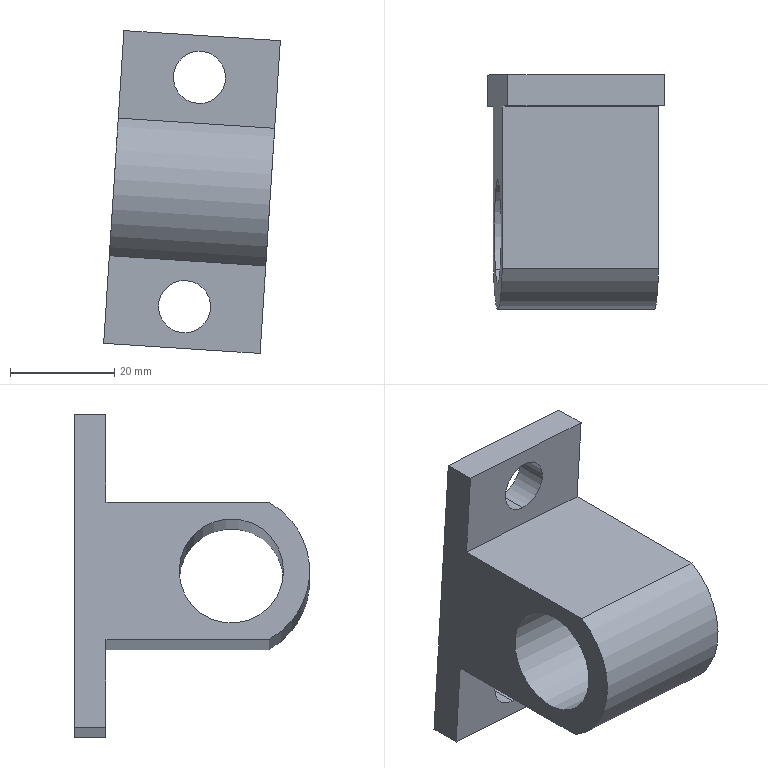Component | SolidWorks | X-AxisBallScrewSupport2-2 | 1 solid | 16 faces | box 33.82 x 45 x 61.82 mm | volume 29524 mm3 | plane 9 | cylinder 7 | commonest cylinder face diameters 10 x4 20 x2 30 x1
build123d program:
from build123d import *

# Parameters (mm, degrees)
SKETCH1_R               = 10
BOSS_EXTRUDE1_DEPTH     = 30
CUT_EXTRUDE1_DEPTH      = 832.191
CUT_EXTRUDE1_DEPTH_BACK = 832.191
CUT_EXTRUDE2_DEPTH      = 779.008
CUT_EXTRUDE2_DEPTH_BACK = 779.008
SKETCH5_R               = 5


with BuildPart() as part:
    # Sketch1 → Boss-Extrude1 (new body)
    with BuildSketch(Plane.XY):
        with BuildLine():
            Line((-298.984, -768.399), (-258.103, -724.481))
            Line((-258.103, -724.481), (-262.495, -720.393))
            Line((-262.495, -720.393), (-296.724, -711.484))
            ThreePointArc((-296.724, -711.484), (-311.482, -715.78), (-314.711, -730.807))
            Line((-314.711, -730.807), (-303.376, -764.311))
            Line((-303.376, -764.311), (-298.984, -768.399))
        make_face()
        with Locations((-300.503, -726)):
            Circle(SKETCH1_R, mode=Mode.SUBTRACT)
    extrude(amount=-BOSS_EXTRUDE1_DEPTH)

    # Sketch4 → Cut-Extrude1 (cut, two sides: drawn at the far end of the back side and taken through both)
    with BuildSketch(Plane(origin=(0, 0, -30), x_dir=(-1, 0, 0), z_dir=(0, 0, -1)).offset(-CUT_EXTRUDE1_DEPTH_BACK)):
        Polygon((314.711, -730.807), (291.929, -752.014), (303.376, -764.311), align=None)
        Polygon((296.724, -711.484), (273.942, -732.69), (262.495, -720.393), align=None)
    extrude(amount=CUT_EXTRUDE1_DEPTH + CUT_EXTRUDE1_DEPTH_BACK, mode=Mode.SUBTRACT)

    # Sketch5 → Cut-Extrude2 (cut, two sides: drawn at the far end of the back side and taken through both)
    with BuildSketch(Plane(origin=(218.636, -203.516, 0), x_dir=(0, 0, 1), z_dir=(-0.732, 0.6813, 0)).offset(-CUT_EXTRUDE2_DEPTH_BACK)):
        with Locations(Location((-15, -714.151, 0), (0, 0, 90))):
            Circle(SKETCH5_R)
        with Locations(Location((-15, -758.151, 0), (0, 0, 90))):
            Circle(SKETCH5_R)
    extrude(amount=CUT_EXTRUDE2_DEPTH + CUT_EXTRUDE2_DEPTH_BACK, mode=Mode.SUBTRACT)


solid = part.part

# Placed as in the assembly
solid = solid.moved(Location((207.979, -970.699, 434.364), (180, 86.288, -47.051)))
STEP:
#1=CARTESIAN_POINT('',(5.654,-26.22,-12.843));
#2=VERTEX_POINT('',#1);
#3=CARTESIAN_POINT('',(5.679,-26.22,-12.45));
#4=VERTEX_POINT('',#3);
#5=CARTESIAN_POINT('',(5.666,-26.22,-12.647));
#6=DIRECTION('',(0.,1.,0.));
#7=DIRECTION('',(0.06474,-0.,0.9979));
#8=AXIS2_PLACEMENT_3D('',#5,#6,#7);
#9=CIRCLE('',#8,0.1969);
#10=EDGE_CURVE('',#2,#4,#9,.T.);
#11=ORIENTED_EDGE('',*,*,#10,.T.);
#12=CARTESIAN_POINT('',(5.679,-26.457,-12.45));
#13=VERTEX_POINT('',#12);
#14=CARTESIAN_POINT('',(5.679,-25.042,-12.45));
#15=DIRECTION('',(0.,-1.,0.));
#16=VECTOR('',#15,39.37);
#17=LINE('',#14,#16);
#18=EDGE_CURVE('',#4,#13,#17,.T.);
#19=ORIENTED_EDGE('',*,*,#18,.T.);
#20=CARTESIAN_POINT('',(5.654,-26.457,-12.843));
#21=VERTEX_POINT('',#20);
#22=CARTESIAN_POINT('',(5.666,-26.457,-12.647));
#23=DIRECTION('',(0.,1.,0.));
#24=DIRECTION('',(0.06474,-0.,0.9979));
#25=AXIS2_PLACEMENT_3D('',#22,#23,#24);
#26=CIRCLE('',#25,0.1969);
#27=EDGE_CURVE('',#21,#13,#26,.T.);
#28=ORIENTED_EDGE('',*,*,#27,.F.);
#29=CARTESIAN_POINT('',(5.654,-25.042,-12.843));
#30=DIRECTION('',(0.,-1.,0.));
#31=VECTOR('',#30,39.37);
#32=LINE('',#29,#31);
#33=EDGE_CURVE('',#2,#21,#32,.T.);
#34=ORIENTED_EDGE('',*,*,#33,.F.);
#35=EDGE_LOOP('',(#11,#19,#28,#34));
#36=FACE_OUTER_BOUND('',#35,.T.);
#37=CARTESIAN_POINT('',(5.666,-25.042,-12.647));
#38=DIRECTION('',(0.,-1.,0.));
#39=DIRECTION('',(-0.06474,0.,-0.9979));
#40=AXIS2_PLACEMENT_3D('',#37,#38,#39);
#41=CYLINDRICAL_SURFACE('',#40,0.1969);
#42=ADVANCED_FACE('',(#36),#41,.F.);
#43=CARTESIAN_POINT('',(5.766,-26.22,-11.114));
#44=VERTEX_POINT('',#43);
#45=CARTESIAN_POINT('',(5.791,-26.22,-10.722));
#46=VERTEX_POINT('',#45);
#47=CARTESIAN_POINT('',(5.779,-26.22,-10.918));
#48=DIRECTION('',(0.,1.,0.));
#49=DIRECTION('',(0.06474,-0.,0.9979));
#50=AXIS2_PLACEMENT_3D('',#47,#48,#49);
#51=CIRCLE('',#50,0.1969);
#52=EDGE_CURVE('',#44,#46,#51,.T.);
#53=ORIENTED_EDGE('',*,*,#52,.T.);
#54=CARTESIAN_POINT('',(5.791,-26.457,-10.722));
#55=VERTEX_POINT('',#54);
#56=CARTESIAN_POINT('',(5.791,-25.042,-10.722));
#57=DIRECTION('',(0.,-1.,0.));
#58=VECTOR('',#57,39.37);
#59=LINE('',#56,#58);
#60=EDGE_CURVE('',#46,#55,#59,.T.);
#61=ORIENTED_EDGE('',*,*,#60,.T.);
#62=CARTESIAN_POINT('',(5.766,-26.457,-11.114));
#63=VERTEX_POINT('',#62);
#64=CARTESIAN_POINT('',(5.779,-26.457,-10.918));
#65=DIRECTION('',(0.,1.,0.));
#66=DIRECTION('',(0.06474,0.,0.9979));
#67=AXIS2_PLACEMENT_3D('',#64,#65,#66);
#68=CIRCLE('',#67,0.1969);
#69=EDGE_CURVE('',#63,#55,#68,.T.);
#70=ORIENTED_EDGE('',*,*,#69,.F.);
#71=CARTESIAN_POINT('',(5.766,-25.042,-11.114));
#72=DIRECTION('',(0.,-1.,0.));
#73=VECTOR('',#72,39.37);
#74=LINE('',#71,#73);
#75=EDGE_CURVE('',#44,#63,#74,.T.);
#76=ORIENTED_EDGE('',*,*,#75,.F.);
#77=EDGE_LOOP('',(#53,#61,#70,#76));
#78=FACE_OUTER_BOUND('',#77,.T.);
#79=CARTESIAN_POINT('',(5.779,-25.042,-10.918));
#80=DIRECTION('',(0.,-1.,0.));
#81=DIRECTION('',(-0.06474,0.,-0.9979));
#82=AXIS2_PLACEMENT_3D('',#79,#80,#81);
#83=CYLINDRICAL_SURFACE('',#82,0.1969);
#84=ADVANCED_FACE('',(#78),#83,.F.);
#85=CARTESIAN_POINT('',(5.116,-27.69,-12.012));
#86=VERTEX_POINT('',#85);
#87=CARTESIAN_POINT('',(5.151,-27.113,-11.476));
#88=VERTEX_POINT('',#87);
#89=CARTESIAN_POINT('',(5.133,-27.402,-11.744));
#90=DIRECTION('',(0.9979,0.,-0.06474));
#91=DIRECTION('',(0.04411,0.732,0.6799));
#92=AXIS2_PLACEMENT_3D('',#89,#90,#91);
#93=CIRCLE('',#92,0.3937);
#94=EDGE_CURVE('',#86,#88,#93,.T.);
#95=ORIENTED_EDGE('',*,*,#94,.F.);
#96=CARTESIAN_POINT('',(6.294,-27.69,-12.088));
#97=VERTEX_POINT('',#96);
#98=CARTESIAN_POINT('',(5.116,-27.69,-12.012));
#99=DIRECTION('',(0.9979,0.,-0.06474));
#100=VECTOR('',#99,39.37);
#101=LINE('',#98,#100);
#102=EDGE_CURVE('',#86,#97,#101,.T.);
#103=ORIENTED_EDGE('',*,*,#102,.T.);
#104=CARTESIAN_POINT('',(6.329,-27.113,-11.553));
#105=VERTEX_POINT('',#104);
#106=CARTESIAN_POINT('',(6.312,-27.402,-11.821));
#107=DIRECTION('',(0.9979,0.,-0.06474));
#108=DIRECTION('',(0.04411,0.732,0.6799));
#109=AXIS2_PLACEMENT_3D('',#106,#107,#108);
#110=CIRCLE('',#109,0.3937);
#111=EDGE_CURVE('',#97,#105,#110,.T.);
#112=ORIENTED_EDGE('',*,*,#111,.T.);
#113=CARTESIAN_POINT('',(5.151,-27.113,-11.476));
#114=DIRECTION('',(0.9979,0.,-0.06474));
#115=VECTOR('',#114,39.37);
#116=LINE('',#113,#115);
#117=EDGE_CURVE('',#88,#105,#116,.T.);
#118=ORIENTED_EDGE('',*,*,#117,.F.);
#119=EDGE_LOOP('',(#95,#103,#112,#118));
#120=FACE_OUTER_BOUND('',#119,.T.);
#121=CARTESIAN_POINT('',(5.133,-27.402,-11.744));
#122=DIRECTION('',(0.9979,0.,-0.06474));
#123=DIRECTION('',(0.04411,0.732,0.6799));
#124=AXIS2_PLACEMENT_3D('',#121,#122,#123);
#125=CYLINDRICAL_SURFACE('',#124,0.3937);
#126=ADVANCED_FACE('',(#120),#125,.F.);
#127=CARTESIAN_POINT('',(6.235,-26.22,-12.999));
#128=VERTEX_POINT('',#127);
#129=CARTESIAN_POINT('',(6.235,-26.457,-12.999));
#130=VERTEX_POINT('',#129);
#131=CARTESIAN_POINT('',(6.235,-38.216,-12.999));
#132=DIRECTION('',(-0.,-1.,-0.));
#133=VECTOR('',#132,39.37);
#134=LINE('',#131,#133);
#135=EDGE_CURVE('',#128,#130,#134,.T.);
#136=ORIENTED_EDGE('',*,*,#135,.T.);
#137=CARTESIAN_POINT('',(5.057,-26.457,-12.923));
#138=VERTEX_POINT('',#137);
#139=CARTESIAN_POINT('',(5.057,-26.457,-12.923));
#140=DIRECTION('',(0.9979,0.,-0.06474));
#141=VECTOR('',#140,39.37);
#142=LINE('',#139,#141);
#143=EDGE_CURVE('',#138,#130,#142,.T.);
#144=ORIENTED_EDGE('',*,*,#143,.F.);
#145=CARTESIAN_POINT('',(5.057,-26.22,-12.923));
#146=VERTEX_POINT('',#145);
#147=CARTESIAN_POINT('',(5.057,-38.216,-12.923));
#148=DIRECTION('',(-0.,-1.,-0.));
#149=VECTOR('',#148,39.37);
#150=LINE('',#147,#149);
#151=EDGE_CURVE('',#146,#138,#150,.T.);
#152=ORIENTED_EDGE('',*,*,#151,.F.);
#153=CARTESIAN_POINT('',(5.057,-26.22,-12.923));
#154=DIRECTION('',(0.9979,0.,-0.06474));
#155=VECTOR('',#154,39.37);
#156=LINE('',#153,#155);
#157=EDGE_CURVE('',#146,#128,#156,.T.);
#158=ORIENTED_EDGE('',*,*,#157,.T.);
#159=EDGE_LOOP('',(#136,#144,#152,#158));
#160=FACE_OUTER_BOUND('',#159,.T.);
#161=CARTESIAN_POINT('',(5.057,-38.216,-12.923));
#162=DIRECTION('',(0.06474,-0.,0.9979));
#163=DIRECTION('',(-0.,-1.,-0.));
#164=AXIS2_PLACEMENT_3D('',#161,#162,#163);
#165=PLANE('',#164);
#166=ADVANCED_FACE('',(#160),#165,.F.);
#167=CARTESIAN_POINT('',(6.345,-27.682,-11.302));
#168=VERTEX_POINT('',#167);
#169=CARTESIAN_POINT('',(6.278,-27.682,-12.339));
#170=VERTEX_POINT('',#169);
#171=CARTESIAN_POINT('',(6.312,-27.402,-11.821));
#172=DIRECTION('',(0.9979,0.,-0.06474));
#173=DIRECTION('',(0.04411,0.732,0.6799));
#174=AXIS2_PLACEMENT_3D('',#171,#172,#173);
#175=CIRCLE('',#174,0.5906);
#176=EDGE_CURVE('',#168,#170,#175,.T.);
#177=ORIENTED_EDGE('',*,*,#176,.F.);
#178=CARTESIAN_POINT('',(5.167,-27.682,-11.226));
#179=VERTEX_POINT('',#178);
#180=CARTESIAN_POINT('',(5.167,-27.682,-11.226));
#181=DIRECTION('',(0.9979,0.,-0.06474));
#182=VECTOR('',#181,39.37);
#183=LINE('',#180,#182);
#184=EDGE_CURVE('',#179,#168,#183,.T.);
#185=ORIENTED_EDGE('',*,*,#184,.F.);
#186=CARTESIAN_POINT('',(5.1,-27.682,-12.263));
#187=VERTEX_POINT('',#186);
#188=CARTESIAN_POINT('',(5.133,-27.402,-11.744));
#189=DIRECTION('',(0.9979,0.,-0.06474));
#190=DIRECTION('',(0.04411,0.732,0.6799));
#191=AXIS2_PLACEMENT_3D('',#188,#189,#190);
#192=CIRCLE('',#191,0.5906);
#193=EDGE_CURVE('',#179,#187,#192,.T.);
#194=ORIENTED_EDGE('',*,*,#193,.T.);
#195=CARTESIAN_POINT('',(5.1,-27.682,-12.263));
#196=DIRECTION('',(0.9979,0.,-0.06474));
#197=VECTOR('',#196,39.37);
#198=LINE('',#195,#197);
#199=EDGE_CURVE('',#187,#170,#198,.T.);
#200=ORIENTED_EDGE('',*,*,#199,.T.);
#201=EDGE_LOOP('',(#177,#185,#194,#200));
#202=FACE_OUTER_BOUND('',#201,.T.);
#203=CARTESIAN_POINT('',(5.133,-27.402,-11.744));
#204=DIRECTION('',(0.9979,0.,-0.06474));
#205=DIRECTION('',(0.04411,0.732,0.6799));
#206=AXIS2_PLACEMENT_3D('',#203,#204,#205);
#207=CYLINDRICAL_SURFACE('',#206,0.5906);
#208=ADVANCED_FACE('',(#202),#207,.T.);
#209=CARTESIAN_POINT('',(6.388,-26.22,-10.642));
#210=VERTEX_POINT('',#209);
#211=CARTESIAN_POINT('',(6.388,-26.457,-10.642));
#212=VERTEX_POINT('',#211);
#213=CARTESIAN_POINT('',(6.388,-38.216,-10.642));
#214=DIRECTION('',(0.,-1.,0.));
#215=VECTOR('',#214,39.37);
#216=LINE('',#213,#215);
#217=EDGE_CURVE('',#210,#212,#216,.T.);
#218=ORIENTED_EDGE('',*,*,#217,.F.);
#219=CARTESIAN_POINT('',(5.21,-26.22,-10.565));
#220=VERTEX_POINT('',#219);
#221=CARTESIAN_POINT('',(5.21,-26.22,-10.565));
#222=DIRECTION('',(0.9979,0.,-0.06474));
#223=VECTOR('',#222,39.37);
#224=LINE('',#221,#223);
#225=EDGE_CURVE('',#220,#210,#224,.T.);
#226=ORIENTED_EDGE('',*,*,#225,.F.);
#227=CARTESIAN_POINT('',(5.21,-26.457,-10.565));
#228=VERTEX_POINT('',#227);
#229=CARTESIAN_POINT('',(5.21,-38.216,-10.565));
#230=DIRECTION('',(0.,-1.,0.));
#231=VECTOR('',#230,39.37);
#232=LINE('',#229,#231);
#233=EDGE_CURVE('',#220,#228,#232,.T.);
#234=ORIENTED_EDGE('',*,*,#233,.T.);
#235=CARTESIAN_POINT('',(5.21,-26.457,-10.565));
#236=DIRECTION('',(0.9979,0.,-0.06474));
#237=VECTOR('',#236,39.37);
#238=LINE('',#235,#237);
#239=EDGE_CURVE('',#228,#212,#238,.T.);
#240=ORIENTED_EDGE('',*,*,#239,.T.);
#241=EDGE_LOOP('',(#218,#226,#234,#240));
#242=FACE_OUTER_BOUND('',#241,.T.);
#243=CARTESIAN_POINT('',(5.21,-38.216,-10.565));
#244=DIRECTION('',(0.06474,0.,0.9979));
#245=DIRECTION('',(0.,-1.,0.));
#246=AXIS2_PLACEMENT_3D('',#243,#244,#245);
#247=PLANE('',#246);
#248=ADVANCED_FACE('',(#242),#247,.T.);
#249=ORIENTED_EDGE('',*,*,#10,.F.);
#250=CARTESIAN_POINT('',(5.666,-26.22,-12.647));
#251=DIRECTION('',(0.,1.,0.));
#252=DIRECTION('',(0.06474,-0.,0.9979));
#253=AXIS2_PLACEMENT_3D('',#250,#251,#252);
#254=CIRCLE('',#253,0.1969);
#255=EDGE_CURVE('',#4,#2,#254,.T.);
#256=ORIENTED_EDGE('',*,*,#255,.F.);
#257=EDGE_LOOP('',(#249,#256));
#258=FACE_BOUND('',#257,.T.);
#259=ORIENTED_EDGE('',*,*,#52,.F.);
#260=CARTESIAN_POINT('',(5.779,-26.22,-10.918));
#261=DIRECTION('',(0.,1.,0.));
#262=DIRECTION('',(0.06474,-0.,0.9979));
#263=AXIS2_PLACEMENT_3D('',#260,#261,#262);
#264=CIRCLE('',#263,0.1969);
#265=EDGE_CURVE('',#46,#44,#264,.T.);
#266=ORIENTED_EDGE('',*,*,#265,.F.);
#267=EDGE_LOOP('',(#259,#266));
#268=FACE_BOUND('',#267,.T.);
#269=CARTESIAN_POINT('',(8.188,-26.22,17.101));
#270=DIRECTION('',(0.06474,-0.,0.9979));
#271=VECTOR('',#270,39.37);
#272=LINE('',#269,#271);
#273=EDGE_CURVE('',#128,#210,#272,.T.);
#274=ORIENTED_EDGE('',*,*,#273,.F.);
#275=ORIENTED_EDGE('',*,*,#157,.F.);
#276=CARTESIAN_POINT('',(7.01,-26.22,17.177));
#277=DIRECTION('',(0.06474,-0.,0.9979));
#278=VECTOR('',#277,39.37);
#279=LINE('',#276,#278);
#280=EDGE_CURVE('',#146,#220,#279,.T.);
#281=ORIENTED_EDGE('',*,*,#280,.T.);
#282=ORIENTED_EDGE('',*,*,#225,.T.);
#283=EDGE_LOOP('',(#274,#275,#281,#282));
#284=FACE_OUTER_BOUND('',#283,.T.);
#285=CARTESIAN_POINT('',(7.01,-26.22,17.177));
#286=DIRECTION('',(0.,1.,0.));
#287=DIRECTION('',(0.06474,-0.,0.9979));
#288=AXIS2_PLACEMENT_3D('',#285,#286,#287);
#289=PLANE('',#288);
#290=ADVANCED_FACE('',(#258,#268,#284),#289,.T.);
#291=ORIENTED_EDGE('',*,*,#102,.F.);
#292=CARTESIAN_POINT('',(5.133,-27.402,-11.744));
#293=DIRECTION('',(0.9979,0.,-0.06474));
#294=DIRECTION('',(0.04411,0.732,0.6799));
#295=AXIS2_PLACEMENT_3D('',#292,#293,#294);
#296=CIRCLE('',#295,0.3937);
#297=EDGE_CURVE('',#88,#86,#296,.T.);
#298=ORIENTED_EDGE('',*,*,#297,.F.);
#299=ORIENTED_EDGE('',*,*,#117,.T.);
#300=CARTESIAN_POINT('',(6.312,-27.402,-11.821));
#301=DIRECTION('',(0.9979,0.,-0.06474));
#302=DIRECTION('',(0.04411,0.732,0.6799));
#303=AXIS2_PLACEMENT_3D('',#300,#301,#302);
#304=CIRCLE('',#303,0.3937);
#305=EDGE_CURVE('',#105,#97,#304,.T.);
#306=ORIENTED_EDGE('',*,*,#305,.T.);
#307=EDGE_LOOP('',(#291,#298,#299,#306));
#308=FACE_OUTER_BOUND('',#307,.T.);
#309=CARTESIAN_POINT('',(5.133,-27.402,-11.744));
#310=DIRECTION('',(0.9979,0.,-0.06474));
#311=DIRECTION('',(0.04411,0.732,0.6799));
#312=AXIS2_PLACEMENT_3D('',#309,#310,#311);
#313=CYLINDRICAL_SURFACE('',#312,0.3937);
#314=ADVANCED_FACE('',(#308),#313,.F.);
#315=CARTESIAN_POINT('',(5.167,-26.457,-11.226));
#316=VERTEX_POINT('',#315);
#317=CARTESIAN_POINT('',(5.167,-38.216,-11.226));
#318=DIRECTION('',(0.,1.,0.));
#319=VECTOR('',#318,39.37);
#320=LINE('',#317,#319);
#321=EDGE_CURVE('',#179,#316,#320,.T.);
#322=ORIENTED_EDGE('',*,*,#321,.T.);
#323=CARTESIAN_POINT('',(7.01,-26.457,17.177));
#324=DIRECTION('',(0.06474,-0.,0.9979));
#325=VECTOR('',#324,39.37);
#326=LINE('',#323,#325);
#327=EDGE_CURVE('',#316,#228,#326,.T.);
#328=ORIENTED_EDGE('',*,*,#327,.T.);
#329=ORIENTED_EDGE('',*,*,#233,.F.);
#330=ORIENTED_EDGE('',*,*,#280,.F.);
#331=ORIENTED_EDGE('',*,*,#151,.T.);
#332=CARTESIAN_POINT('',(5.1,-26.457,-12.263));
#333=VERTEX_POINT('',#332);
#334=CARTESIAN_POINT('',(7.01,-26.457,17.177));
#335=DIRECTION('',(0.06474,-0.,0.9979));
#336=VECTOR('',#335,39.37);
#337=LINE('',#334,#336);
#338=EDGE_CURVE('',#138,#333,#337,.T.);
#339=ORIENTED_EDGE('',*,*,#338,.T.);
#340=CARTESIAN_POINT('',(5.1,-38.216,-12.263));
#341=DIRECTION('',(-0.,-1.,-0.));
#342=VECTOR('',#341,39.37);
#343=LINE('',#340,#342);
#344=EDGE_CURVE('',#333,#187,#343,.T.);
#345=ORIENTED_EDGE('',*,*,#344,.T.);
#346=ORIENTED_EDGE('',*,*,#193,.F.);
#347=EDGE_LOOP('',(#322,#328,#329,#330,#331,#339,#345,#346));
#348=FACE_OUTER_BOUND('',#347,.T.);
#349=ORIENTED_EDGE('',*,*,#297,.T.);
#350=ORIENTED_EDGE('',*,*,#94,.T.);
#351=EDGE_LOOP('',(#349,#350));
#352=FACE_BOUND('',#351,.T.);
#353=CARTESIAN_POINT('',(7.01,-38.216,17.177));
#354=DIRECTION('',(0.9979,0.,-0.06474));
#355=DIRECTION('',(0.04411,0.732,0.6799));
#356=AXIS2_PLACEMENT_3D('',#353,#354,#355);
#357=PLANE('',#356);
#358=ADVANCED_FACE('',(#348,#352),#357,.F.);
#359=CARTESIAN_POINT('',(6.345,-26.457,-11.302));
#360=VERTEX_POINT('',#359);
#361=CARTESIAN_POINT('',(6.388,-26.457,-10.642));
#362=DIRECTION('',(-0.06474,0.,-0.9979));
#363=VECTOR('',#362,39.37);
#364=LINE('',#361,#363);
#365=EDGE_CURVE('',#212,#360,#364,.T.);
#366=ORIENTED_EDGE('',*,*,#365,.T.);
#367=CARTESIAN_POINT('',(6.345,-27.682,-11.302));
#368=DIRECTION('',(-0.,-1.,-0.));
#369=VECTOR('',#368,39.37);
#370=LINE('',#367,#369);
#371=EDGE_CURVE('',#360,#168,#370,.T.);
#372=ORIENTED_EDGE('',*,*,#371,.T.);
#373=ORIENTED_EDGE('',*,*,#176,.T.);
#374=CARTESIAN_POINT('',(6.278,-26.457,-12.339));
#375=VERTEX_POINT('',#374);
#376=CARTESIAN_POINT('',(6.278,-27.682,-12.339));
#377=DIRECTION('',(0.,1.,0.));
#378=VECTOR('',#377,39.37);
#379=LINE('',#376,#378);
#380=EDGE_CURVE('',#170,#375,#379,.T.);
#381=ORIENTED_EDGE('',*,*,#380,.T.);
#382=CARTESIAN_POINT('',(6.278,-26.457,-12.339));
#383=DIRECTION('',(-0.06474,0.,-0.9979));
#384=VECTOR('',#383,39.37);
#385=LINE('',#382,#384);
#386=EDGE_CURVE('',#375,#130,#385,.T.);
#387=ORIENTED_EDGE('',*,*,#386,.T.);
#388=ORIENTED_EDGE('',*,*,#135,.F.);
#389=ORIENTED_EDGE('',*,*,#273,.T.);
#390=ORIENTED_EDGE('',*,*,#217,.T.);
#391=EDGE_LOOP('',(#366,#372,#373,#381,#387,#388,#389,#390));
#392=FACE_OUTER_BOUND('',#391,.T.);
#393=ORIENTED_EDGE('',*,*,#305,.F.);
#394=ORIENTED_EDGE('',*,*,#111,.F.);
#395=EDGE_LOOP('',(#393,#394));
#396=FACE_BOUND('',#395,.T.);
#397=CARTESIAN_POINT('',(8.188,-38.216,17.101));
#398=DIRECTION('',(0.9979,0.,-0.06474));
#399=DIRECTION('',(0.04411,0.732,0.6799));
#400=AXIS2_PLACEMENT_3D('',#397,#398,#399);
#401=PLANE('',#400);
#402=ADVANCED_FACE('',(#392,#396),#401,.T.);
#403=ORIENTED_EDGE('',*,*,#27,.T.);
#404=CARTESIAN_POINT('',(5.666,-26.457,-12.647));
#405=DIRECTION('',(0.,1.,0.));
#406=DIRECTION('',(0.06474,-0.,0.9979));
#407=AXIS2_PLACEMENT_3D('',#404,#405,#406);
#408=CIRCLE('',#407,0.1969);
#409=EDGE_CURVE('',#13,#21,#408,.T.);
#410=ORIENTED_EDGE('',*,*,#409,.T.);
#411=EDGE_LOOP('',(#403,#410));
#412=FACE_BOUND('',#411,.T.);
#413=ORIENTED_EDGE('',*,*,#143,.T.);
#414=ORIENTED_EDGE('',*,*,#386,.F.);
#415=CARTESIAN_POINT('',(6.278,-26.457,-12.339));
#416=DIRECTION('',(-0.9979,-0.,0.06474));
#417=VECTOR('',#416,39.37);
#418=LINE('',#415,#417);
#419=EDGE_CURVE('',#375,#333,#418,.T.);
#420=ORIENTED_EDGE('',*,*,#419,.T.);
#421=ORIENTED_EDGE('',*,*,#338,.F.);
#422=EDGE_LOOP('',(#413,#414,#420,#421));
#423=FACE_OUTER_BOUND('',#422,.T.);
#424=CARTESIAN_POINT('',(6.278,-26.457,-12.339));
#425=DIRECTION('',(0.,1.,0.));
#426=DIRECTION('',(0.06474,-0.,0.9979));
#427=AXIS2_PLACEMENT_3D('',#424,#425,#426);
#428=PLANE('',#427);
#429=ADVANCED_FACE('',(#412,#423),#428,.F.);
#430=ORIENTED_EDGE('',*,*,#419,.F.);
#431=ORIENTED_EDGE('',*,*,#380,.F.);
#432=ORIENTED_EDGE('',*,*,#199,.F.);
#433=ORIENTED_EDGE('',*,*,#344,.F.);
#434=EDGE_LOOP('',(#430,#431,#432,#433));
#435=FACE_OUTER_BOUND('',#434,.T.);
#436=CARTESIAN_POINT('',(6.278,-27.682,-12.339));
#437=DIRECTION('',(0.06474,-0.,0.9979));
#438=DIRECTION('',(-0.,-1.,-0.));
#439=AXIS2_PLACEMENT_3D('',#436,#437,#438);
#440=PLANE('',#439);
#441=ADVANCED_FACE('',(#435),#440,.F.);
#442=ORIENTED_EDGE('',*,*,#69,.T.);
#443=CARTESIAN_POINT('',(5.779,-26.457,-10.918));
#444=DIRECTION('',(0.,1.,0.));
#445=DIRECTION('',(0.06474,0.,0.9979));
#446=AXIS2_PLACEMENT_3D('',#443,#444,#445);
#447=CIRCLE('',#446,0.1969);
#448=EDGE_CURVE('',#55,#63,#447,.T.);
#449=ORIENTED_EDGE('',*,*,#448,.T.);
#450=EDGE_LOOP('',(#442,#449));
#451=FACE_BOUND('',#450,.T.);
#452=CARTESIAN_POINT('',(6.345,-26.457,-11.302));
#453=DIRECTION('',(-0.9979,-0.,0.06474));
#454=VECTOR('',#453,39.37);
#455=LINE('',#452,#454);
#456=EDGE_CURVE('',#360,#316,#455,.T.);
#457=ORIENTED_EDGE('',*,*,#456,.F.);
#458=ORIENTED_EDGE('',*,*,#365,.F.);
#459=ORIENTED_EDGE('',*,*,#239,.F.);
#460=ORIENTED_EDGE('',*,*,#327,.F.);
#461=EDGE_LOOP('',(#457,#458,#459,#460));
#462=FACE_OUTER_BOUND('',#461,.T.);
#463=CARTESIAN_POINT('',(6.388,-26.457,-10.642));
#464=DIRECTION('',(0.,1.,0.));
#465=DIRECTION('',(0.06474,-0.,0.9979));
#466=AXIS2_PLACEMENT_3D('',#463,#464,#465);
#467=PLANE('',#466);
#468=ADVANCED_FACE('',(#451,#462),#467,.F.);
#469=ORIENTED_EDGE('',*,*,#184,.T.);
#470=ORIENTED_EDGE('',*,*,#371,.F.);
#471=ORIENTED_EDGE('',*,*,#456,.T.);
#472=ORIENTED_EDGE('',*,*,#321,.F.);
#473=EDGE_LOOP('',(#469,#470,#471,#472));
#474=FACE_OUTER_BOUND('',#473,.T.);
#475=CARTESIAN_POINT('',(6.345,-27.682,-11.302));
#476=DIRECTION('',(-0.06474,0.,-0.9979));
#477=DIRECTION('',(0.,1.,0.));
#478=AXIS2_PLACEMENT_3D('',#475,#476,#477);
#479=PLANE('',#478);
#480=ADVANCED_FACE('',(#474),#479,.F.);
#481=ORIENTED_EDGE('',*,*,#60,.F.);
#482=ORIENTED_EDGE('',*,*,#265,.T.);
#483=ORIENTED_EDGE('',*,*,#75,.T.);
#484=ORIENTED_EDGE('',*,*,#448,.F.);
#485=EDGE_LOOP('',(#481,#482,#483,#484));
#486=FACE_OUTER_BOUND('',#485,.T.);
#487=CARTESIAN_POINT('',(5.779,-25.042,-10.918));
#488=DIRECTION('',(0.,-1.,0.));
#489=DIRECTION('',(-0.06474,0.,-0.9979));
#490=AXIS2_PLACEMENT_3D('',#487,#488,#489);
#491=CYLINDRICAL_SURFACE('',#490,0.1969);
#492=ADVANCED_FACE('',(#486),#491,.F.);
#493=ORIENTED_EDGE('',*,*,#18,.F.);
#494=ORIENTED_EDGE('',*,*,#255,.T.);
#495=ORIENTED_EDGE('',*,*,#33,.T.);
#496=ORIENTED_EDGE('',*,*,#409,.F.);
#497=EDGE_LOOP('',(#493,#494,#495,#496));
#498=FACE_OUTER_BOUND('',#497,.T.);
#499=CARTESIAN_POINT('',(5.666,-25.042,-12.647));
#500=DIRECTION('',(0.,-1.,0.));
#501=DIRECTION('',(-0.06474,0.,-0.9979));
#502=AXIS2_PLACEMENT_3D('',#499,#500,#501);
#503=CYLINDRICAL_SURFACE('',#502,0.1969);
#504=ADVANCED_FACE('',(#498),#503,.F.);
#505=CLOSED_SHELL('',(#42,#84,#126,#166,#208,#248,#290,#314,#358,#402,#429,#441,#468,#480,#492,#504));
#506=MANIFOLD_SOLID_BREP('',#505);
#507=CARTESIAN_POINT('',(0.,0.,0.));
#508=DIRECTION('',(0.,0.,1.));
#509=DIRECTION('',(1.,0.,0.));
#510=AXIS2_PLACEMENT_3D('',#507,#508,#509);
#511=(LENGTH_UNIT()NAMED_UNIT(*)SI_UNIT($,.METRE.));
#512=LENGTH_MEASURE_WITH_UNIT(LENGTH_MEASURE(0.0254),#511);
#513=DIMENSIONAL_EXPONENTS(1.,0.,0.,0.,0.,0.,0.);
#514=(CONVERSION_BASED_UNIT('',#512)LENGTH_UNIT()NAMED_UNIT(#513));
#515=UNCERTAINTY_MEASURE_WITH_UNIT(LENGTH_MEASURE(0.00001),#514,'','');
#516=(NAMED_UNIT(*)PLANE_ANGLE_UNIT()SI_UNIT($,.RADIAN.));
#517=(NAMED_UNIT(*)SI_UNIT($,.STERADIAN.)SOLID_ANGLE_UNIT());
#518=(GEOMETRIC_REPRESENTATION_CONTEXT(3)GLOBAL_UNCERTAINTY_ASSIGNED_CONTEXT((#515))GLOBAL_UNIT_ASSIGNED_CONTEXT((#514,#516,#517))REPRESENTATION_CONTEXT('',''));
#519=ADVANCED_BREP_SHAPE_REPRESENTATION('',(#506,#510),#518);
#520=COLOUR_RGB('',0.7922,0.8196,0.9333);
#521=FILL_AREA_STYLE_COLOUR('',#520);
#522=FILL_AREA_STYLE('',(#521));
#523=SURFACE_STYLE_FILL_AREA(#522);
#524=SURFACE_SIDE_STYLE('',(#523));
#525=SURFACE_STYLE_USAGE(.BOTH.,#524);
#526=PRESENTATION_STYLE_ASSIGNMENT((#525));
#527=STYLED_ITEM('',(#526),#506);
#528=PRESENTATION_LAYER_ASSIGNMENT('','',(#527));
#529=(LENGTH_UNIT()NAMED_UNIT(*)SI_UNIT($,.METRE.));
#530=LENGTH_MEASURE_WITH_UNIT(LENGTH_MEASURE(0.0254),#529);
#531=DIMENSIONAL_EXPONENTS(1.,0.,0.,0.,0.,0.,0.);
#532=(CONVERSION_BASED_UNIT('',#530)LENGTH_UNIT()NAMED_UNIT(#531));
#533=UNCERTAINTY_MEASURE_WITH_UNIT(LENGTH_MEASURE(0.00001),#532,'','');
#534=(NAMED_UNIT(*)PLANE_ANGLE_UNIT()SI_UNIT($,.RADIAN.));
#535=(NAMED_UNIT(*)SI_UNIT($,.STERADIAN.)SOLID_ANGLE_UNIT());
#536=(GEOMETRIC_REPRESENTATION_CONTEXT(3)GLOBAL_UNCERTAINTY_ASSIGNED_CONTEXT((#533))GLOBAL_UNIT_ASSIGNED_CONTEXT((#532,#534,#535))REPRESENTATION_CONTEXT('',''));
#537=MECHANICAL_DESIGN_GEOMETRIC_PRESENTATION_REPRESENTATION('',(#527),#536);